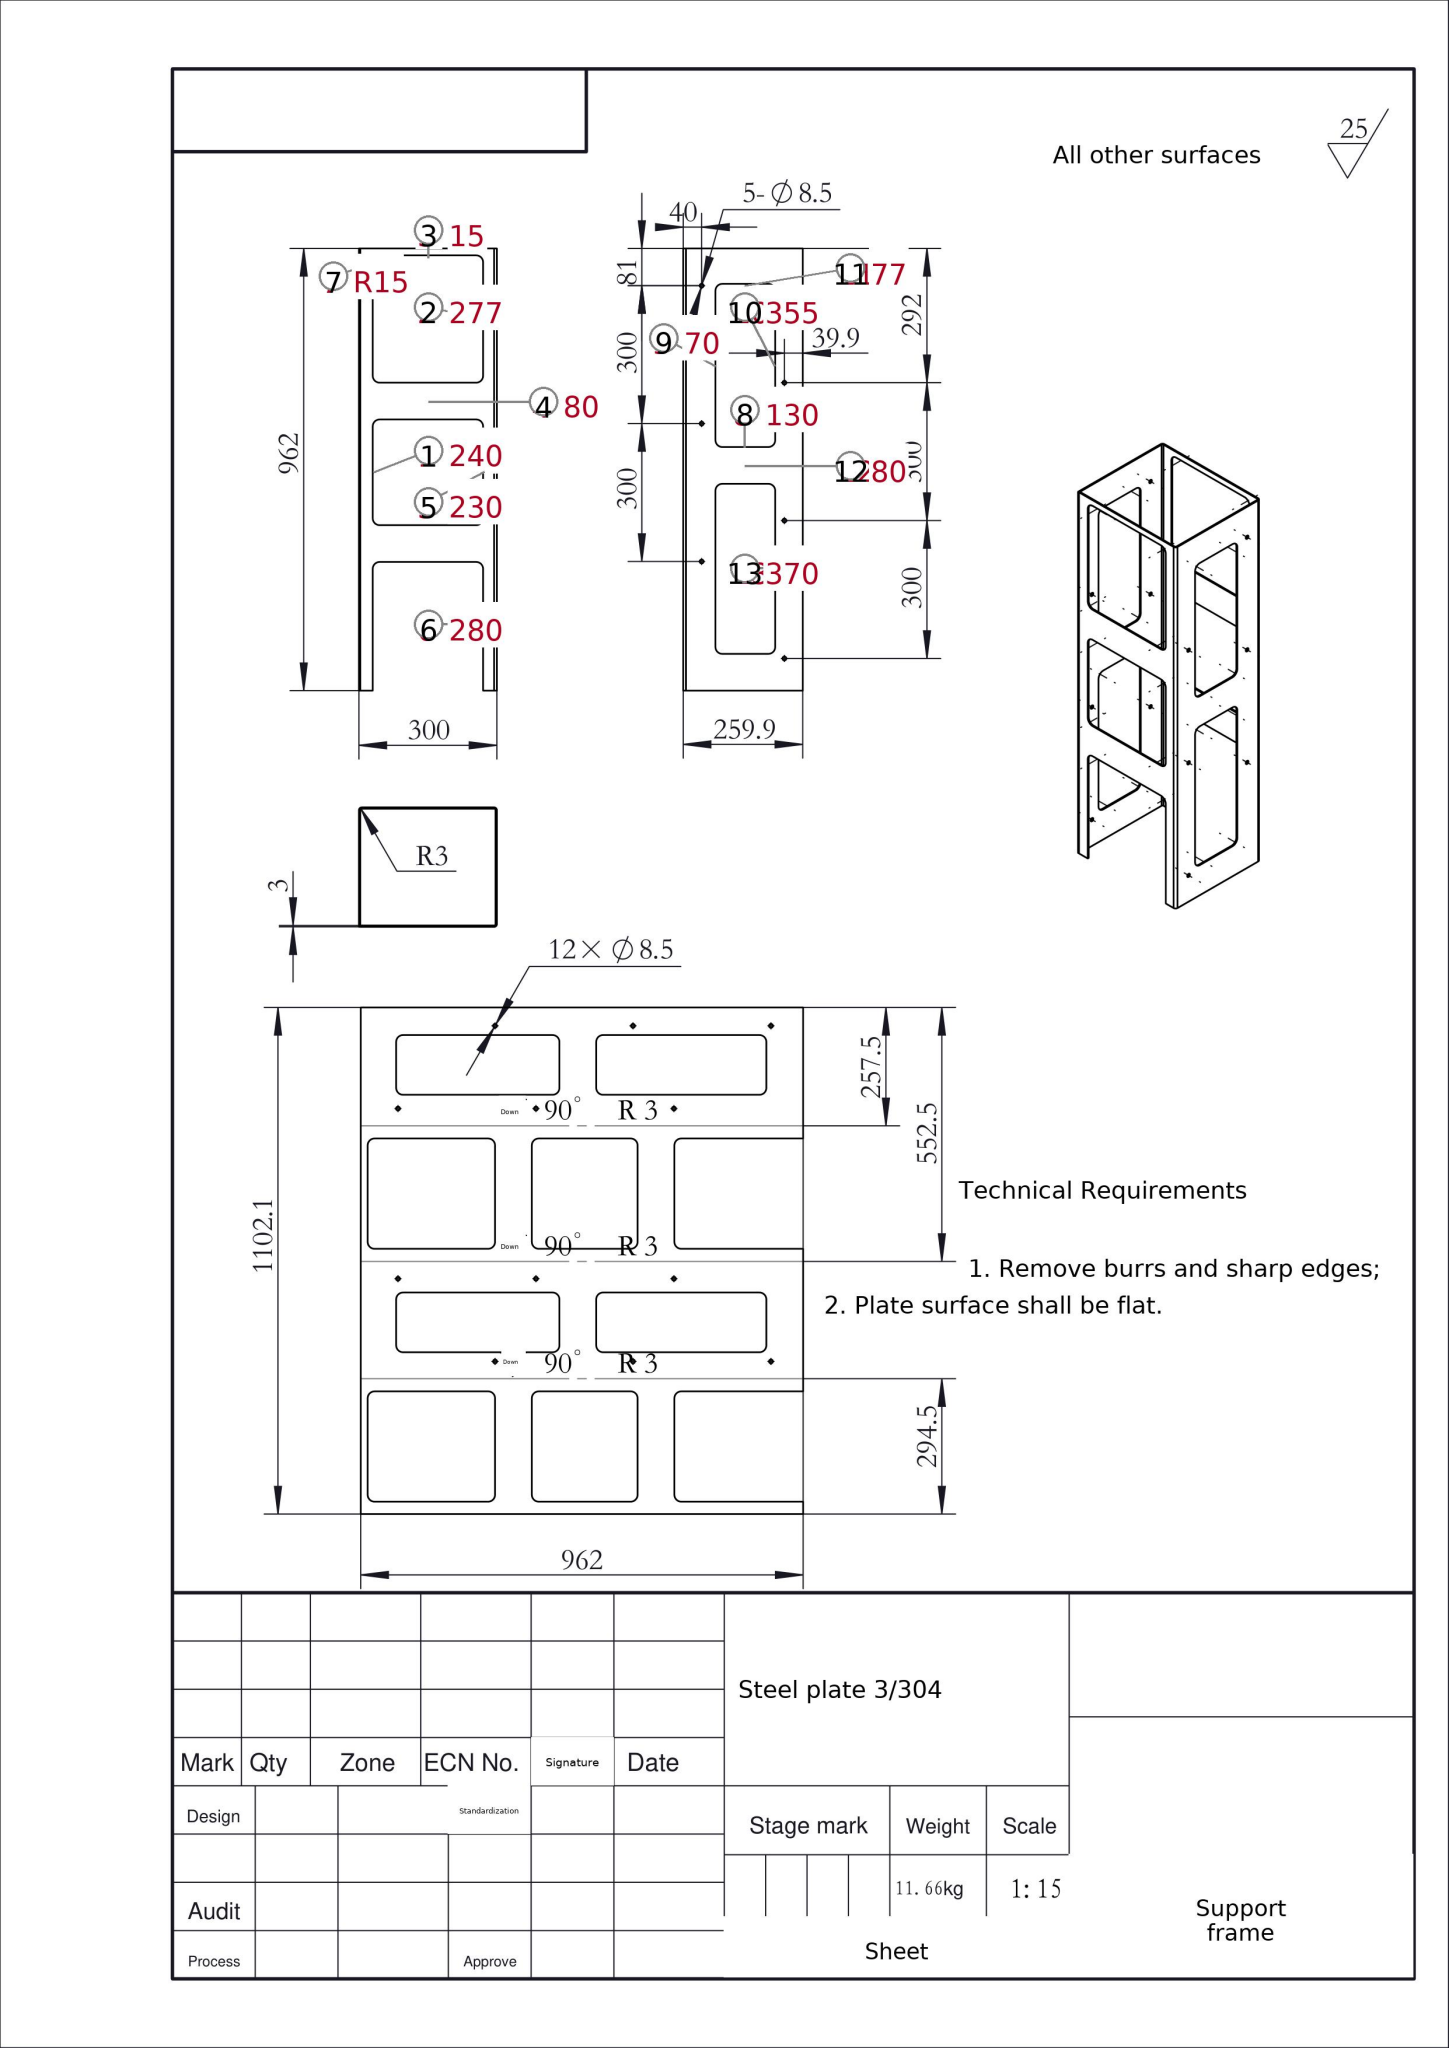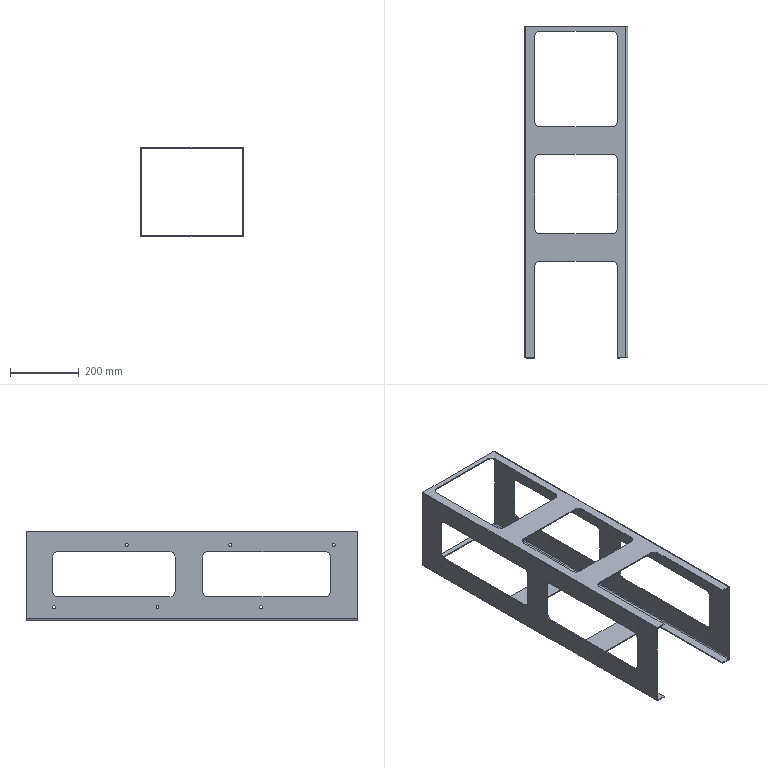Part | SolidWorks | mm | material Steel plate 3/304 | 1 solid | 130 faces | box 300 x 962 x 260 mm | volume 1484950 mm3 | cylinder 66 | plane 64 | commonest cylinder face diameters 30 x36 8.5 x24 6 x3 12 x3